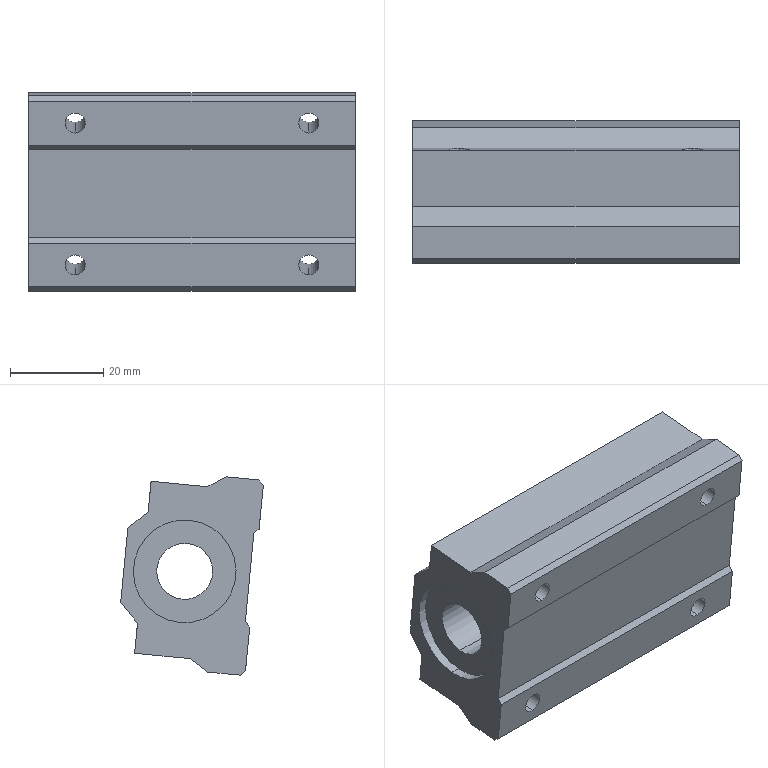Component | SolidWorks | InnerDiameter12Slider(ExtendedVersion)-1 | 1 solid | 36 faces | box 70 x 30.54 x 42.47 mm | volume 59350 mm3 | plane 22 | cylinder 14 | commonest cylinder face diameters 4.3 x8 22 x4 12 x2 | material Aluminum Oxide
build123d program:
from build123d import *

# Parameters (mm, degrees)
SKETCH1_R           = 6
BOSS_EXTRUDE1_DEPTH = 70
SKETCH2_R           = 11
CUT_EXTRUDE1_DEPTH  = 2
CUT_EXTRUDE2_START  = -2
SKETCH3_R           = 11
CUT_EXTRUDE2_DEPTH  = 2
SKETCH4_R           = 2.15
CUT_EXTRUDE3_DEPTH  = 79.262


with BuildPart() as part:
    # Sketch1 → Boss-Extrude1 (new body)
    with BuildSketch(Plane(origin=(0, 0, 0), x_dir=(0, 0, -1), z_dir=(1, 0, 0))):
        Polygon((-21, -7), (-18.5, -3), (-18.5, 9), (-12, 9), (-8, 13), (8, 13), (12, 9), (18.5, 9), (18.5, -3), (21, -7), (21, -13.962), (19.962, -15), (10.538, -15), (9.5, -13.962), (-9.5, -13.962), (-10.538, -15), (-19.962, -15), (-21, -13.962), align=None)
        Circle(SKETCH1_R, mode=Mode.SUBTRACT)
    extrude(amount=BOSS_EXTRUDE1_DEPTH)

    # Sketch2 → Cut-Extrude1 (cut)
    with BuildSketch(Plane(origin=(70, 0, 0), x_dir=(0, 0, -1), z_dir=(1, 0, 0))):
        Circle(SKETCH2_R)
    extrude(amount=-CUT_EXTRUDE1_DEPTH, mode=Mode.SUBTRACT)

    # Sketch3 → Cut-Extrude2 (cut)
    with BuildSketch(Plane.ZY.offset(CUT_EXTRUDE2_START)):
        with Locations(Location((0, 0, 0), (0, 0, 180))):
            Circle(SKETCH3_R)
    extrude(amount=CUT_EXTRUDE2_DEPTH, mode=Mode.SUBTRACT)

    # Sketch4 → Cut-Extrude3 (cut, through all)
    with BuildSketch(Plane.XZ.offset(15)):
        with Locations(Location((10, 15.25, 0), (0, 0, 270))):
            Circle(SKETCH4_R)
        with Locations(Location((60, 15.25, 0), (0, 0, 270))):
            Circle(SKETCH4_R)
        with Locations(Location((10, -15.25, 0), (0, 0, 270))):
            Circle(SKETCH4_R)
        with Locations(Location((60, -15.25, 0), (0, 0, 270))):
            Circle(SKETCH4_R)
    extrude(amount=-CUT_EXTRUDE3_DEPTH, mode=Mode.SUBTRACT)


solid = part.part

# Placed as in the assembly
solid = solid.moved(Location((-270.938, 15.116, 349), (5.481, 0, 0)))